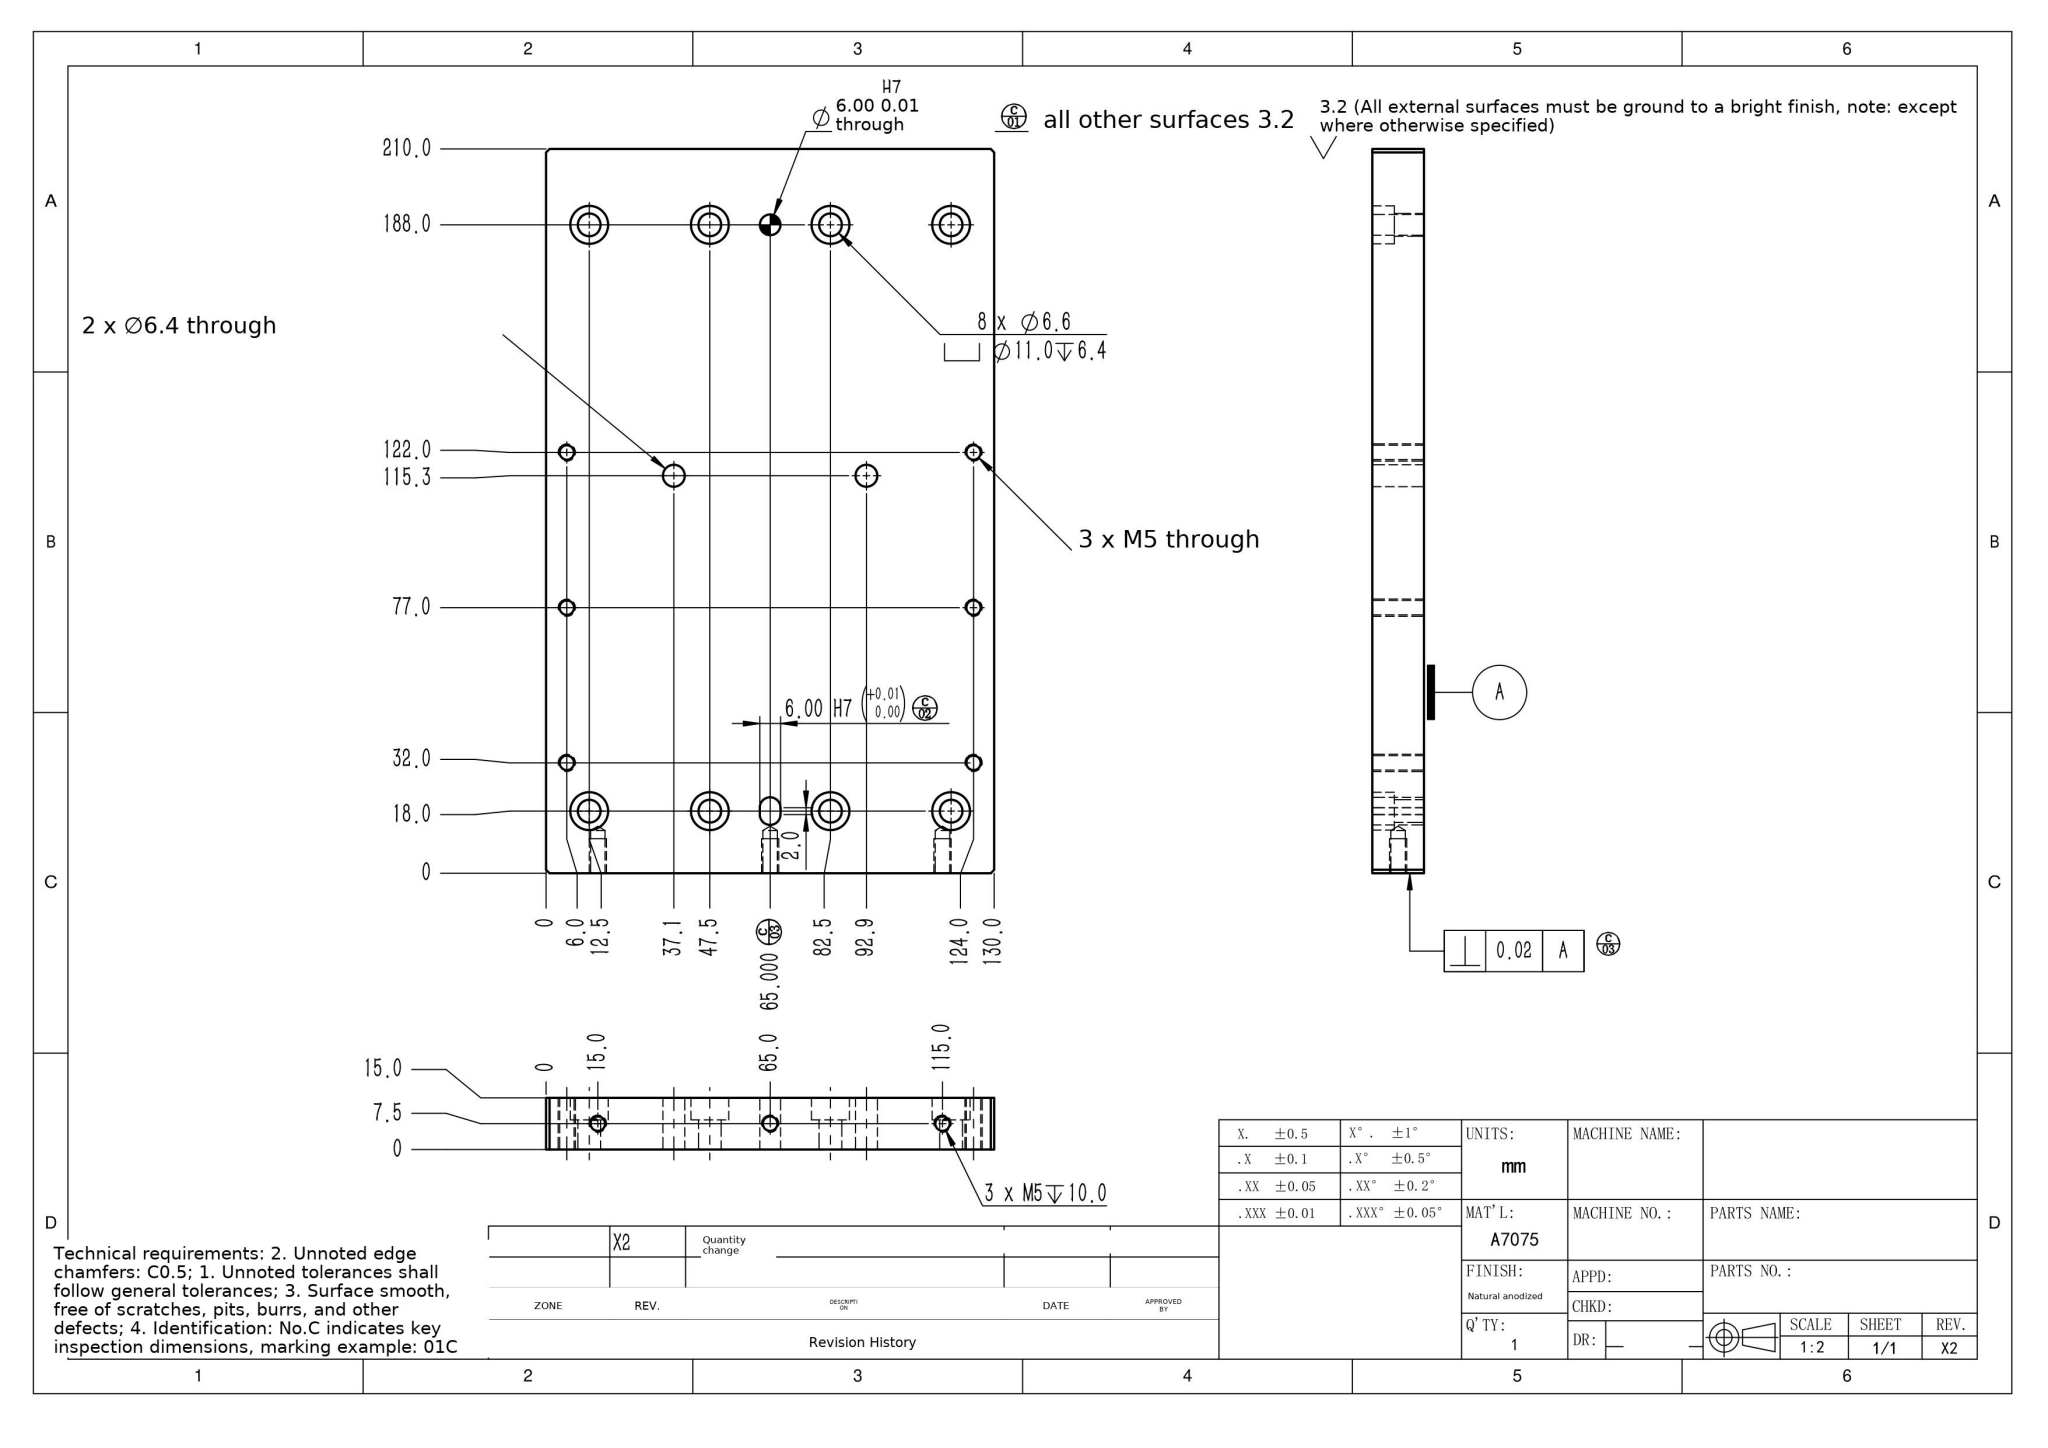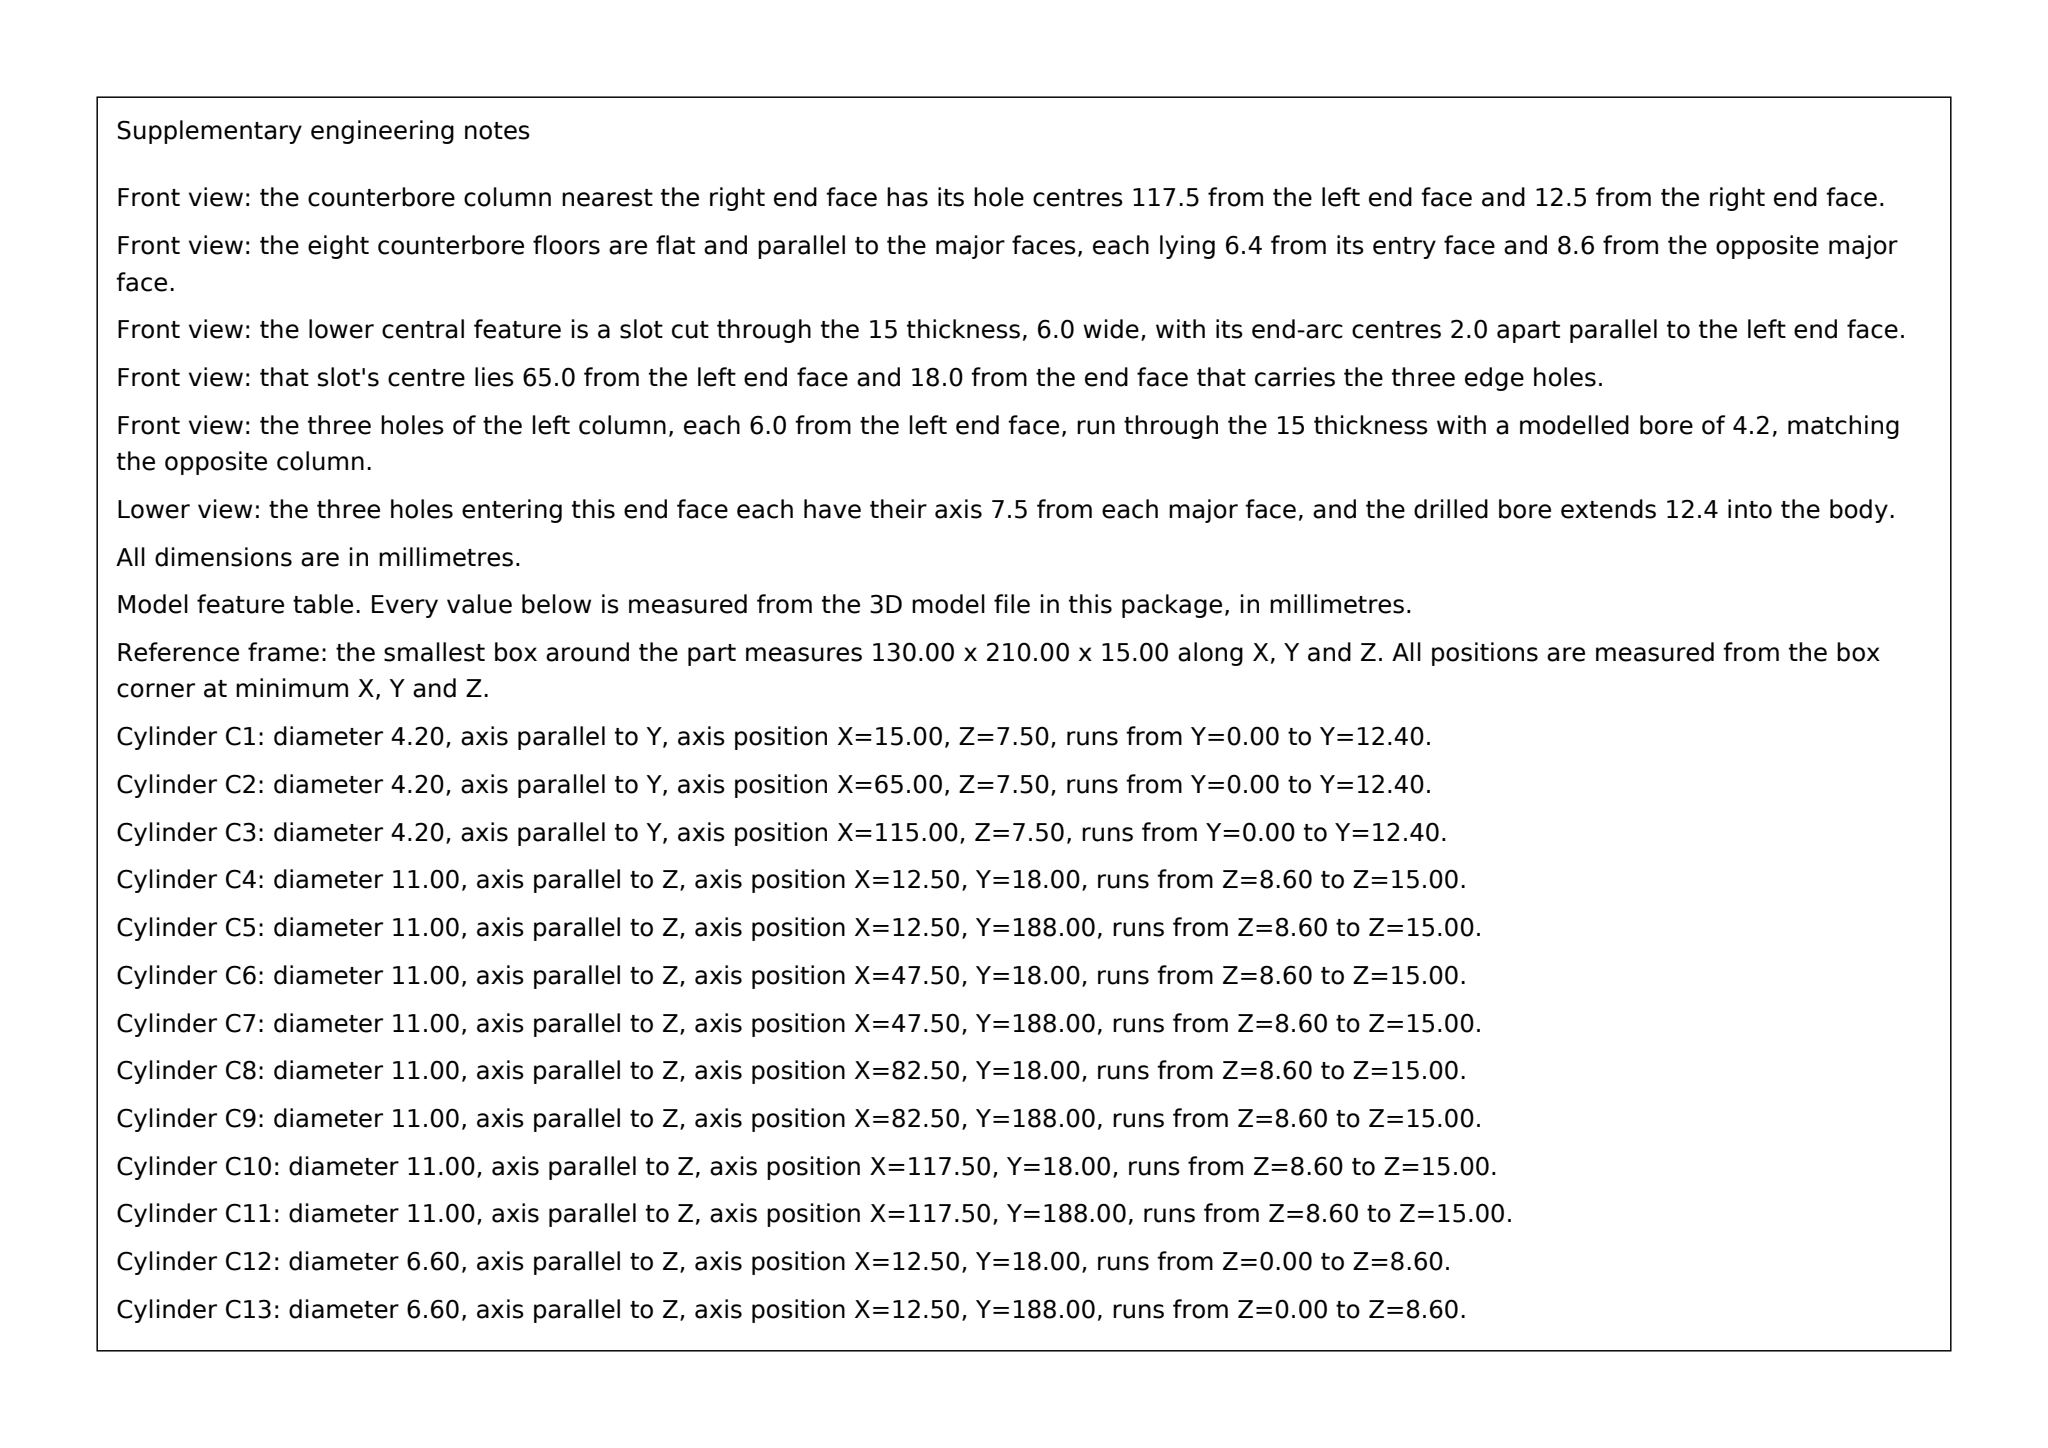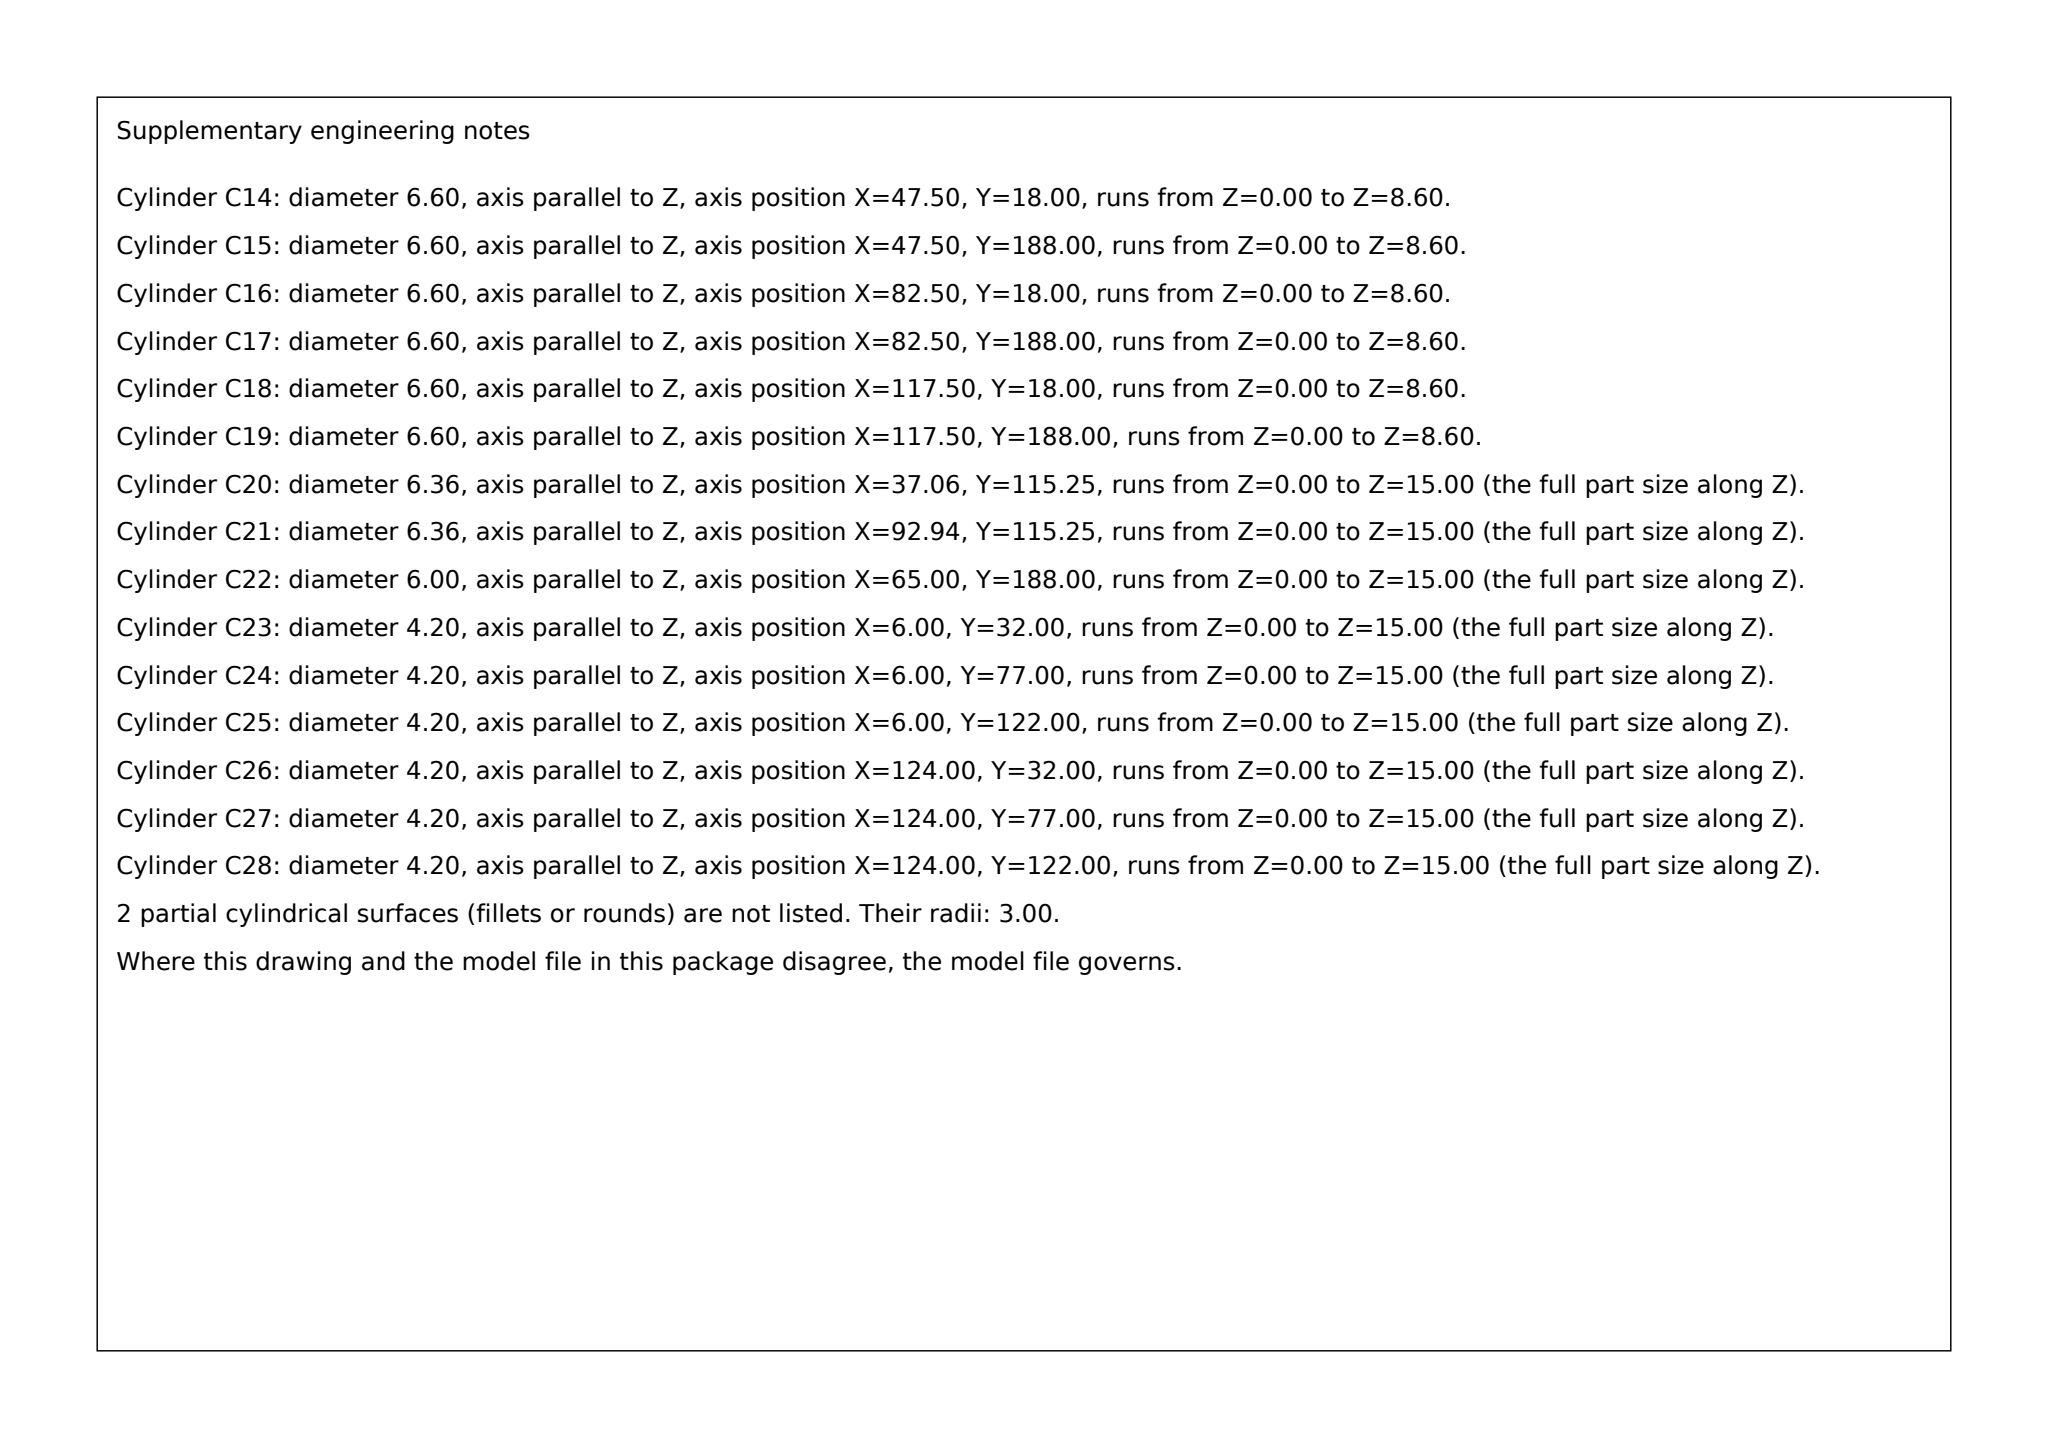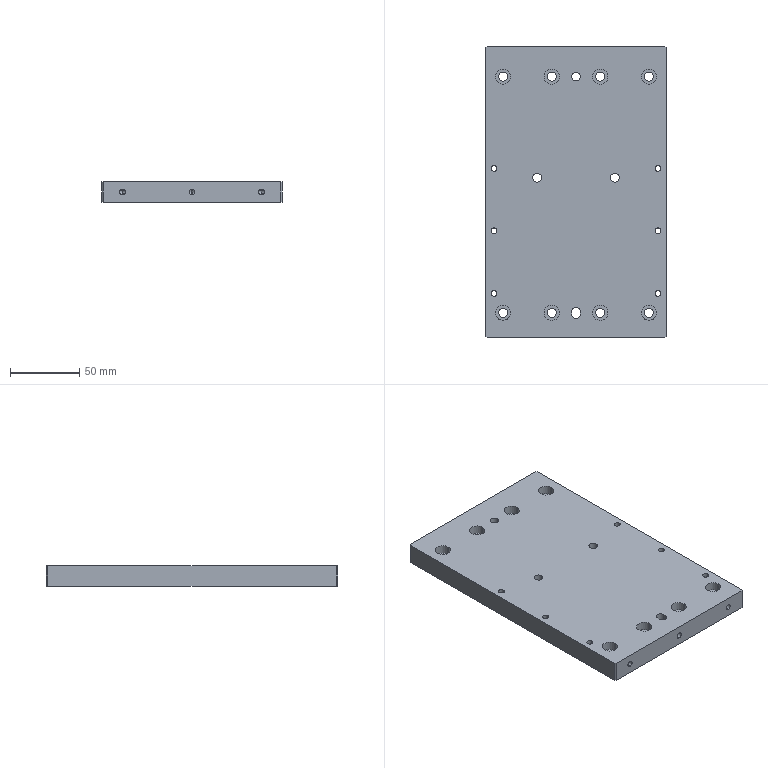Part | SolidWorks | mm | 1 solid | 84 faces | box 130 x 210 x 15 mm | volume 398492 mm3 | cylinder 58 | plane 20 | cone 6 | commonest cylinder face diameters 4.2 x18 11 x16 6.6 x16 6 x4 6.35 x4
build123d program:
from build123d import *

# Parameters (mm, degrees)
SKETCH1_W                                       = 130
SKETCH1_H                                       = 210
BOSS_EXTRUDE1_DEPTH                             = 7.5
M5_TAPPED_HOLE2_D                               = 4.2
M5_TAPPED_HOLE2_DEPTH                           = 12.4
M5_TAPPED_HOLE2_TIP                             = 1.262
M6_HEX_SOCKET_HEAD_CAP_SCREW_CBORE1_D           = 6.6
M6_HEX_SOCKET_HEAD_CAP_SCREW_CBORE1_CBORE_D     = 11
M6_HEX_SOCKET_HEAD_CAP_SCREW_CBORE1_CBORE_DEPTH = 6.4
SKETCH8_R                                       = 3.175
CUT_EXTRUDE1_DEPTH                              = 125.399
M5_TAPPED_HOLE1_D                               = 4.2
SKETCH11_R                                      = 3
CUT_EXTRUDE2_DEPTH                              = 125.399
CHAMFER1_SIZE                                   = 1


with BuildPart() as part:
    # Sketch1 → Boss-Extrude1 (new, symmetric)
    with BuildSketch(Plane.XY):
        Rectangle(SKETCH1_W, SKETCH1_H)
    extrude(amount=BOSS_EXTRUDE1_DEPTH, both=True)

    # M5 Tapped Hole2
    with Locations(Plane(origin=(0, -105, 0), x_dir=(-1, 0, 0), z_dir=(0, -1, 0))):
        with Locations((0, 0), (50, 0), (-50, 0)):
            Hole(M5_TAPPED_HOLE2_D / 2, depth=M5_TAPPED_HOLE2_DEPTH)
            with Locations((0, 0, -(M5_TAPPED_HOLE2_DEPTH + M5_TAPPED_HOLE2_TIP / 2))):  # 118° drill point
                Cone(0, M5_TAPPED_HOLE2_D / 2, M5_TAPPED_HOLE2_TIP, mode=Mode.SUBTRACT)

    # M6 Hex Socket Head Cap Screw CBORE1 (through all)
    with Locations(Plane.XY.offset(7.5)):
        with Locations((17.5, -87), (-52.5, -87), (52.5, -87), (17.5, 83), (-17.5, 83), (-52.5, 83), (52.5, 83), (-17.5, -87)):
            CounterBoreHole(M6_HEX_SOCKET_HEAD_CAP_SCREW_CBORE1_D / 2, M6_HEX_SOCKET_HEAD_CAP_SCREW_CBORE1_CBORE_D / 2, M6_HEX_SOCKET_HEAD_CAP_SCREW_CBORE1_CBORE_DEPTH)

    # Sketch8 → Cut-Extrude1 (cut, through all)
    with BuildSketch(Plane.XY.offset(7.5)):
        with Locations((27.94, 10.25)):
            Circle(SKETCH8_R)
        with Locations((-27.94, 10.25)):
            Circle(SKETCH8_R)
    extrude(amount=-CUT_EXTRUDE1_DEPTH, mode=Mode.SUBTRACT)

    # M5 Tapped Hole1 (through all)
    with Locations(Plane.XY.offset(7.5)):
        with Locations((-59, 17), (-59, -28), (-59, -73)):
            m5_tapped_hole1 = Hole(M5_TAPPED_HOLE1_D / 2)

    # Mirror1: M5 Tapped Hole1 across plane
    add(m5_tapped_hole1.mirror(Plane(origin=(0, 0, 0), x_dir=(0, 0, 1), z_dir=(1, 0, 0))), mode=Mode.SUBTRACT)

    # Sketch11 → Cut-Extrude2 (cut, through all)
    with BuildSketch(Plane.XY.offset(7.5)):
        with Locations((0, 83)):
            Circle(SKETCH11_R)
        with BuildLine():
            Line((-3, -88), (-3, -86))
            ThreePointArc((-3, -86), (0, -83), (3, -86))
            Line((3, -86), (3, -88))
            ThreePointArc((3, -88), (0, -91), (-3, -88))
        make_face()
    extrude(amount=-CUT_EXTRUDE2_DEPTH, mode=Mode.SUBTRACT)

    # Chamfer1
    chamfer1_edges = [part.edges().sort_by_distance(p)[0] for p in [
        (65, -105, 0),
        (-65, -105, 0),
        (-65, 105, 0),
        (65, 105, 0),
    ]]
    chamfer(chamfer1_edges, length=CHAMFER1_SIZE)


solid = part.part